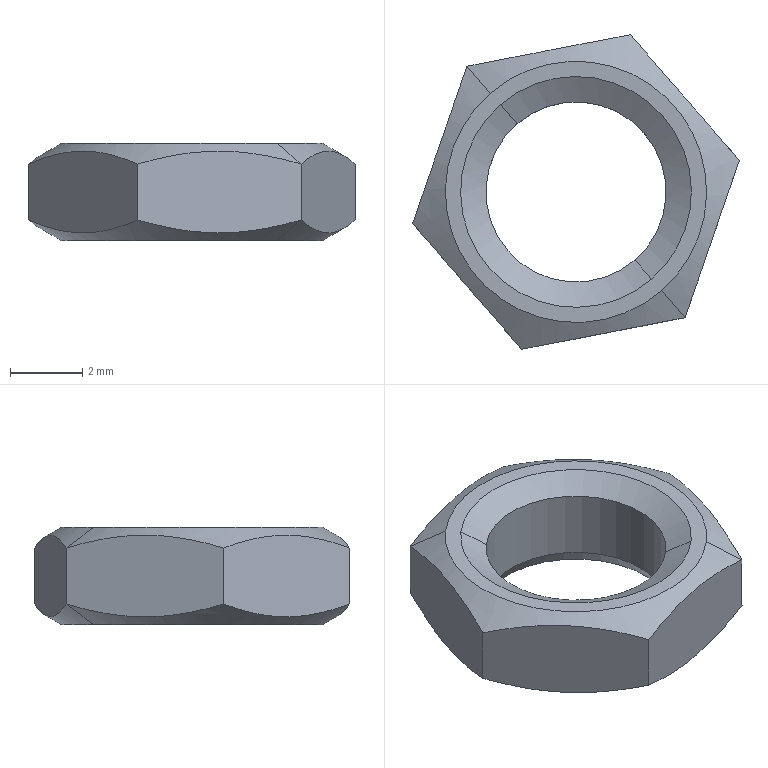Component | SolidWorks | HexThinNutGBT6172.1-M5-1 | 1 solid | 18 faces | box 9.07 x 8.73 x 2.7 mm | volume 88 mm3 | cone 8 | plane 8 | cylinder 2 | commonest cylinder face diameters 5 x2 | material Purchased Part
STEP:
#1=CARTESIAN_POINT('',(-3.125,-0.3253,-0.9055));
#2=VERTEX_POINT('',#1);
#3=CARTESIAN_POINT('',(-2.938,-0.5409,-0.9055));
#4=VERTEX_POINT('',#3);
#5=CARTESIAN_POINT('',(-3.031,-0.4331,-0.9055));
#6=DIRECTION('',(0.,0.,-1.));
#7=DIRECTION('',(0.6555,-0.7552,0.));
#8=AXIS2_PLACEMENT_3D('',#5,#6,#7);
#9=CIRCLE('',#8,0.1427);
#10=EDGE_CURVE('',#2,#4,#9,.T.);
#11=ORIENTED_EDGE('',*,*,#10,.F.);
#12=CARTESIAN_POINT('',(-3.151,-0.2957,-0.8829));
#13=VERTEX_POINT('',#12);
#14=CARTESIAN_POINT('',(-3.151,-0.2956,-0.8828));
#15=DIRECTION('',(-0.5676,0.654,0.5));
#16=VECTOR('',#15,39.37);
#17=LINE('',#14,#16);
#18=EDGE_CURVE('',#2,#13,#17,.T.);
#19=ORIENTED_EDGE('',*,*,#18,.T.);
#20=CARTESIAN_POINT('',(-2.972,-0.2612,-0.8829));
#21=VERTEX_POINT('',#20);
#22=CARTESIAN_POINT('',(-3.151,-0.2957,-0.8829));
#23=CARTESIAN_POINT('',(-3.122,-0.2901,-0.8915));
#24=CARTESIAN_POINT('',(-3.092,-0.2844,-0.897));
#25=CARTESIAN_POINT('',(-3.046,-0.2756,-0.897));
#26=CARTESIAN_POINT('',(-3.031,-0.2726,-0.8957));
#27=CARTESIAN_POINT('',(-3.001,-0.2669,-0.8908));
#28=CARTESIAN_POINT('',(-2.987,-0.264,-0.8872));
#29=CARTESIAN_POINT('',(-2.972,-0.2612,-0.8829));
#30=B_SPLINE_CURVE_WITH_KNOTS('',3,(#22,#23,#24,#25,#26,#27,#28,#29),.UNSPECIFIED.,.F.,.F.,(4,2,2,4),(0.,0.002332,0.003499,0.004665),.UNSPECIFIED.);
#31=EDGE_CURVE('',#13,#21,#30,.T.);
#32=ORIENTED_EDGE('',*,*,#31,.T.);
#33=CARTESIAN_POINT('',(-2.853,-0.3985,-0.8829));
#34=VERTEX_POINT('',#33);
#35=CARTESIAN_POINT('',(-2.972,-0.2612,-0.8829));
#36=CARTESIAN_POINT('',(-2.953,-0.2836,-0.8915));
#37=CARTESIAN_POINT('',(-2.933,-0.3064,-0.897));
#38=CARTESIAN_POINT('',(-2.903,-0.3414,-0.897));
#39=CARTESIAN_POINT('',(-2.892,-0.3531,-0.8957));
#40=CARTESIAN_POINT('',(-2.873,-0.376,-0.8908));
#41=CARTESIAN_POINT('',(-2.863,-0.3873,-0.8872));
#42=CARTESIAN_POINT('',(-2.853,-0.3985,-0.8829));
#43=B_SPLINE_CURVE_WITH_KNOTS('',3,(#35,#36,#37,#38,#39,#40,#41,#42),.UNSPECIFIED.,.F.,.F.,(4,2,2,4),(0.,0.002332,0.003499,0.004665),.UNSPECIFIED.);
#44=EDGE_CURVE('',#21,#34,#43,.T.);
#45=ORIENTED_EDGE('',*,*,#44,.T.);
#46=CARTESIAN_POINT('',(-2.912,-0.5704,-0.8829));
#47=VERTEX_POINT('',#46);
#48=CARTESIAN_POINT('',(-2.853,-0.3985,-0.8829));
#49=CARTESIAN_POINT('',(-2.863,-0.4266,-0.8915));
#50=CARTESIAN_POINT('',(-2.872,-0.4551,-0.897));
#51=CARTESIAN_POINT('',(-2.888,-0.4989,-0.897));
#52=CARTESIAN_POINT('',(-2.893,-0.5135,-0.8957));
#53=CARTESIAN_POINT('',(-2.903,-0.5422,-0.8908));
#54=CARTESIAN_POINT('',(-2.907,-0.5564,-0.8872));
#55=CARTESIAN_POINT('',(-2.912,-0.5704,-0.8829));
#56=B_SPLINE_CURVE_WITH_KNOTS('',3,(#48,#49,#50,#51,#52,#53,#54,#55),.UNSPECIFIED.,.F.,.F.,(4,2,2,4),(0.,0.002332,0.003499,0.004665),.UNSPECIFIED.);
#57=EDGE_CURVE('',#34,#47,#56,.T.);
#58=ORIENTED_EDGE('',*,*,#57,.T.);
#59=CARTESIAN_POINT('',(-2.912,-0.5706,-0.8828));
#60=DIRECTION('',(0.5676,-0.654,0.5));
#61=VECTOR('',#60,39.37);
#62=LINE('',#59,#61);
#63=EDGE_CURVE('',#4,#47,#62,.T.);
#64=ORIENTED_EDGE('',*,*,#63,.F.);
#65=EDGE_LOOP('',(#11,#19,#32,#45,#58,#64));
#66=FACE_OUTER_BOUND('',#65,.T.);
#67=CARTESIAN_POINT('',(-3.031,-0.4331,-0.8828));
#68=DIRECTION('',(0.,0.,1.));
#69=DIRECTION('',(0.6555,-0.7552,0.));
#70=AXIS2_PLACEMENT_3D('',#67,#68,#69);
#71=CONICAL_SURFACE('',#70,0.1821,1.047);
#72=ADVANCED_FACE('',(#66),#71,.T.);
#73=CARTESIAN_POINT('',(-2.967,-0.5074,-0.8903));
#74=VERTEX_POINT('',#73);
#75=CARTESIAN_POINT('',(-3.096,-0.3587,-0.8903));
#76=VERTEX_POINT('',#75);
#77=CARTESIAN_POINT('',(-3.031,-0.4331,-0.8903));
#78=DIRECTION('',(0.,0.,-1.));
#79=DIRECTION('',(-0.6555,0.7552,0.));
#80=AXIS2_PLACEMENT_3D('',#77,#78,#79);
#81=CIRCLE('',#80,0.09843);
#82=EDGE_CURVE('',#74,#76,#81,.T.);
#83=ORIENTED_EDGE('',*,*,#82,.F.);
#84=CARTESIAN_POINT('',(-2.961,-0.514,-0.9055));
#85=VERTEX_POINT('',#84);
#86=CARTESIAN_POINT('',(-2.964,-0.5103,-0.897));
#87=DIRECTION('',(0.3277,-0.3776,-0.866));
#88=VECTOR('',#87,39.37);
#89=LINE('',#86,#88);
#90=EDGE_CURVE('',#74,#85,#89,.T.);
#91=ORIENTED_EDGE('',*,*,#90,.T.);
#92=CARTESIAN_POINT('',(-3.102,-0.3521,-0.9055));
#93=VERTEX_POINT('',#92);
#94=CARTESIAN_POINT('',(-3.031,-0.4331,-0.9055));
#95=DIRECTION('',(0.,0.,1.));
#96=DIRECTION('',(-0.6555,0.7552,0.));
#97=AXIS2_PLACEMENT_3D('',#94,#95,#96);
#98=CIRCLE('',#97,0.1072);
#99=EDGE_CURVE('',#93,#85,#98,.T.);
#100=ORIENTED_EDGE('',*,*,#99,.F.);
#101=CARTESIAN_POINT('',(-3.099,-0.3558,-0.897));
#102=DIRECTION('',(-0.3277,0.3776,-0.866));
#103=VECTOR('',#102,39.37);
#104=LINE('',#101,#103);
#105=EDGE_CURVE('',#76,#93,#104,.T.);
#106=ORIENTED_EDGE('',*,*,#105,.F.);
#107=EDGE_LOOP('',(#83,#91,#100,#106));
#108=FACE_OUTER_BOUND('',#107,.T.);
#109=CARTESIAN_POINT('',(-3.031,-0.4331,-0.897));
#110=DIRECTION('',(0.,0.,-1.));
#111=DIRECTION('',(-0.6555,0.7552,0.));
#112=AXIS2_PLACEMENT_3D('',#109,#110,#111);
#113=CONICAL_SURFACE('',#112,0.1023,0.5236);
#114=ADVANCED_FACE('',(#108),#113,.F.);
#115=ORIENTED_EDGE('',*,*,#82,.T.);
#116=CARTESIAN_POINT('',(-3.096,-0.3587,-0.8152));
#117=VERTEX_POINT('',#116);
#118=CARTESIAN_POINT('',(-3.096,-0.3587,-0.9055));
#119=DIRECTION('',(0.,0.,1.));
#120=VECTOR('',#119,39.37);
#121=LINE('',#118,#120);
#122=EDGE_CURVE('',#76,#117,#121,.T.);
#123=ORIENTED_EDGE('',*,*,#122,.T.);
#124=CARTESIAN_POINT('',(-2.967,-0.5074,-0.8152));
#125=VERTEX_POINT('',#124);
#126=CARTESIAN_POINT('',(-3.031,-0.4331,-0.8152));
#127=DIRECTION('',(0.,0.,-1.));
#128=DIRECTION('',(0.6555,-0.7552,0.));
#129=AXIS2_PLACEMENT_3D('',#126,#127,#128);
#130=CIRCLE('',#129,0.09843);
#131=EDGE_CURVE('',#125,#117,#130,.T.);
#132=ORIENTED_EDGE('',*,*,#131,.F.);
#133=CARTESIAN_POINT('',(-2.967,-0.5074,-0.9055));
#134=DIRECTION('',(0.,0.,1.));
#135=VECTOR('',#134,39.37);
#136=LINE('',#133,#135);
#137=EDGE_CURVE('',#74,#125,#136,.T.);
#138=ORIENTED_EDGE('',*,*,#137,.F.);
#139=EDGE_LOOP('',(#115,#123,#132,#138));
#140=FACE_OUTER_BOUND('',#139,.T.);
#141=CARTESIAN_POINT('',(-3.031,-0.4331,-0.9055));
#142=DIRECTION('',(0.,0.,1.));
#143=DIRECTION('',(0.6555,-0.7552,0.));
#144=AXIS2_PLACEMENT_3D('',#141,#142,#143);
#145=CYLINDRICAL_SURFACE('',#144,0.09843);
#146=ADVANCED_FACE('',(#140),#145,.F.);
#147=CARTESIAN_POINT('',(-3.125,-0.3253,-0.7992));
#148=VERTEX_POINT('',#147);
#149=CARTESIAN_POINT('',(-2.938,-0.5409,-0.7992));
#150=VERTEX_POINT('',#149);
#151=CARTESIAN_POINT('',(-3.031,-0.4331,-0.7992));
#152=DIRECTION('',(0.,0.,-1.));
#153=DIRECTION('',(-0.6555,0.7552,0.));
#154=AXIS2_PLACEMENT_3D('',#151,#152,#153);
#155=CIRCLE('',#154,0.1427);
#156=EDGE_CURVE('',#148,#150,#155,.T.);
#157=ORIENTED_EDGE('',*,*,#156,.T.);
#158=CARTESIAN_POINT('',(-2.912,-0.5704,-0.8218));
#159=VERTEX_POINT('',#158);
#160=CARTESIAN_POINT('',(-2.912,-0.5706,-0.8219));
#161=DIRECTION('',(0.5676,-0.654,-0.5));
#162=VECTOR('',#161,39.37);
#163=LINE('',#160,#162);
#164=EDGE_CURVE('',#150,#159,#163,.T.);
#165=ORIENTED_EDGE('',*,*,#164,.T.);
#166=CARTESIAN_POINT('',(-2.853,-0.3985,-0.8218));
#167=VERTEX_POINT('',#166);
#168=CARTESIAN_POINT('',(-2.853,-0.3985,-0.8218));
#169=CARTESIAN_POINT('',(-2.863,-0.4266,-0.8132));
#170=CARTESIAN_POINT('',(-2.872,-0.4551,-0.8078));
#171=CARTESIAN_POINT('',(-2.888,-0.4989,-0.8077));
#172=CARTESIAN_POINT('',(-2.893,-0.5135,-0.8091));
#173=CARTESIAN_POINT('',(-2.903,-0.5422,-0.814));
#174=CARTESIAN_POINT('',(-2.907,-0.5564,-0.8175));
#175=CARTESIAN_POINT('',(-2.912,-0.5704,-0.8218));
#176=B_SPLINE_CURVE_WITH_KNOTS('',3,(#168,#169,#170,#171,#172,#173,#174,#175),.UNSPECIFIED.,.F.,.F.,(4,2,2,4),(0.,0.002332,0.003499,0.004665),.UNSPECIFIED.);
#177=EDGE_CURVE('',#167,#159,#176,.T.);
#178=ORIENTED_EDGE('',*,*,#177,.F.);
#179=CARTESIAN_POINT('',(-2.972,-0.2612,-0.8218));
#180=VERTEX_POINT('',#179);
#181=CARTESIAN_POINT('',(-2.972,-0.2612,-0.8218));
#182=CARTESIAN_POINT('',(-2.953,-0.2836,-0.8132));
#183=CARTESIAN_POINT('',(-2.933,-0.3064,-0.8078));
#184=CARTESIAN_POINT('',(-2.903,-0.3414,-0.8077));
#185=CARTESIAN_POINT('',(-2.892,-0.3531,-0.8091));
#186=CARTESIAN_POINT('',(-2.873,-0.376,-0.814));
#187=CARTESIAN_POINT('',(-2.863,-0.3873,-0.8175));
#188=CARTESIAN_POINT('',(-2.853,-0.3985,-0.8218));
#189=B_SPLINE_CURVE_WITH_KNOTS('',3,(#181,#182,#183,#184,#185,#186,#187,#188),.UNSPECIFIED.,.F.,.F.,(4,2,2,4),(0.,0.002332,0.003499,0.004665),.UNSPECIFIED.);
#190=EDGE_CURVE('',#180,#167,#189,.T.);
#191=ORIENTED_EDGE('',*,*,#190,.F.);
#192=CARTESIAN_POINT('',(-3.151,-0.2957,-0.8218));
#193=VERTEX_POINT('',#192);
#194=CARTESIAN_POINT('',(-3.151,-0.2957,-0.8218));
#195=CARTESIAN_POINT('',(-3.122,-0.2901,-0.8132));
#196=CARTESIAN_POINT('',(-3.092,-0.2844,-0.8078));
#197=CARTESIAN_POINT('',(-3.046,-0.2756,-0.8077));
#198=CARTESIAN_POINT('',(-3.031,-0.2726,-0.8091));
#199=CARTESIAN_POINT('',(-3.001,-0.2669,-0.814));
#200=CARTESIAN_POINT('',(-2.987,-0.264,-0.8175));
#201=CARTESIAN_POINT('',(-2.972,-0.2612,-0.8218));
#202=B_SPLINE_CURVE_WITH_KNOTS('',3,(#194,#195,#196,#197,#198,#199,#200,#201),.UNSPECIFIED.,.F.,.F.,(4,2,2,4),(0.,0.002332,0.003499,0.004665),.UNSPECIFIED.);
#203=EDGE_CURVE('',#193,#180,#202,.T.);
#204=ORIENTED_EDGE('',*,*,#203,.F.);
#205=CARTESIAN_POINT('',(-3.151,-0.2956,-0.8219));
#206=DIRECTION('',(-0.5676,0.654,-0.5));
#207=VECTOR('',#206,39.37);
#208=LINE('',#205,#207);
#209=EDGE_CURVE('',#148,#193,#208,.T.);
#210=ORIENTED_EDGE('',*,*,#209,.F.);
#211=EDGE_LOOP('',(#157,#165,#178,#191,#204,#210));
#212=FACE_OUTER_BOUND('',#211,.T.);
#213=CARTESIAN_POINT('',(-3.031,-0.4331,-0.8219));
#214=DIRECTION('',(0.,0.,-1.));
#215=DIRECTION('',(-0.6555,0.7552,0.));
#216=AXIS2_PLACEMENT_3D('',#213,#214,#215);
#217=CONICAL_SURFACE('',#216,0.1821,1.047);
#218=ADVANCED_FACE('',(#212),#217,.T.);
#219=ORIENTED_EDGE('',*,*,#131,.T.);
#220=CARTESIAN_POINT('',(-3.114,-0.3378,-0.7992));
#221=VERTEX_POINT('',#220);
#222=CARTESIAN_POINT('',(-3.097,-0.3571,-0.814));
#223=DIRECTION('',(-0.5676,0.654,0.5));
#224=VECTOR('',#223,39.37);
#225=LINE('',#222,#224);
#226=EDGE_CURVE('',#117,#221,#225,.T.);
#227=ORIENTED_EDGE('',*,*,#226,.T.);
#228=CARTESIAN_POINT('',(-2.949,-0.5283,-0.7992));
#229=VERTEX_POINT('',#228);
#230=CARTESIAN_POINT('',(-3.031,-0.4331,-0.7992));
#231=DIRECTION('',(0.,0.,-1.));
#232=DIRECTION('',(-0.6555,0.7552,0.));
#233=AXIS2_PLACEMENT_3D('',#230,#231,#232);
#234=CIRCLE('',#233,0.1261);
#235=EDGE_CURVE('',#229,#221,#234,.T.);
#236=ORIENTED_EDGE('',*,*,#235,.F.);
#237=CARTESIAN_POINT('',(-2.966,-0.509,-0.814));
#238=DIRECTION('',(0.5676,-0.654,0.5));
#239=VECTOR('',#238,39.37);
#240=LINE('',#237,#239);
#241=EDGE_CURVE('',#125,#229,#240,.T.);
#242=ORIENTED_EDGE('',*,*,#241,.F.);
#243=EDGE_LOOP('',(#219,#227,#236,#242));
#244=FACE_OUTER_BOUND('',#243,.T.);
#245=CARTESIAN_POINT('',(-3.031,-0.4331,-0.814));
#246=DIRECTION('',(0.,0.,1.));
#247=DIRECTION('',(0.6555,-0.7552,0.));
#248=AXIS2_PLACEMENT_3D('',#245,#246,#247);
#249=CONICAL_SURFACE('',#248,0.1005,1.047);
#250=ADVANCED_FACE('',(#244),#249,.F.);
#251=CARTESIAN_POINT('',(-3.031,-0.4331,-0.9055));
#252=DIRECTION('',(0.,0.,-1.));
#253=DIRECTION('',(0.6555,-0.7552,0.));
#254=AXIS2_PLACEMENT_3D('',#251,#252,#253);
#255=CIRCLE('',#254,0.1427);
#256=EDGE_CURVE('',#4,#2,#255,.T.);
#257=ORIENTED_EDGE('',*,*,#256,.T.);
#258=ORIENTED_EDGE('',*,*,#10,.T.);
#259=EDGE_LOOP('',(#257,#258));
#260=FACE_OUTER_BOUND('',#259,.T.);
#261=ORIENTED_EDGE('',*,*,#99,.T.);
#262=CARTESIAN_POINT('',(-3.031,-0.4331,-0.9055));
#263=DIRECTION('',(0.,0.,1.));
#264=DIRECTION('',(-0.6555,0.7552,0.));
#265=AXIS2_PLACEMENT_3D('',#262,#263,#264);
#266=CIRCLE('',#265,0.1072);
#267=EDGE_CURVE('',#85,#93,#266,.T.);
#268=ORIENTED_EDGE('',*,*,#267,.T.);
#269=EDGE_LOOP('',(#261,#268));
#270=FACE_BOUND('',#269,.T.);
#271=CARTESIAN_POINT('',(-3.21,-0.4676,-0.9055));
#272=DIRECTION('',(0.,0.,-1.));
#273=DIRECTION('',(-0.6555,0.7552,0.));
#274=AXIS2_PLACEMENT_3D('',#271,#272,#273);
#275=PLANE('',#274);
#276=ADVANCED_FACE('',(#260,#270),#275,.T.);
#277=ORIENTED_EDGE('',*,*,#18,.F.);
#278=ORIENTED_EDGE('',*,*,#256,.F.);
#279=ORIENTED_EDGE('',*,*,#63,.T.);
#280=CARTESIAN_POINT('',(-3.091,-0.605,-0.8829));
#281=VERTEX_POINT('',#280);
#282=CARTESIAN_POINT('',(-2.912,-0.5704,-0.8829));
#283=CARTESIAN_POINT('',(-2.941,-0.576,-0.8915));
#284=CARTESIAN_POINT('',(-2.971,-0.5818,-0.897));
#285=CARTESIAN_POINT('',(-3.017,-0.5906,-0.897));
#286=CARTESIAN_POINT('',(-3.032,-0.5935,-0.8957));
#287=CARTESIAN_POINT('',(-3.062,-0.5993,-0.8908));
#288=CARTESIAN_POINT('',(-3.076,-0.6021,-0.8872));
#289=CARTESIAN_POINT('',(-3.091,-0.605,-0.8829));
#290=B_SPLINE_CURVE_WITH_KNOTS('',3,(#282,#283,#284,#285,#286,#287,#288,#289),.UNSPECIFIED.,.F.,.F.,(4,2,2,4),(0.,0.002332,0.003499,0.004665),.UNSPECIFIED.);
#291=EDGE_CURVE('',#47,#281,#290,.T.);
#292=ORIENTED_EDGE('',*,*,#291,.T.);
#293=CARTESIAN_POINT('',(-3.21,-0.4676,-0.8829));
#294=VERTEX_POINT('',#293);
#295=CARTESIAN_POINT('',(-3.091,-0.605,-0.8829));
#296=CARTESIAN_POINT('',(-3.11,-0.5825,-0.8915));
#297=CARTESIAN_POINT('',(-3.13,-0.5598,-0.897));
#298=CARTESIAN_POINT('',(-3.16,-0.5247,-0.897));
#299=CARTESIAN_POINT('',(-3.171,-0.5131,-0.8957));
#300=CARTESIAN_POINT('',(-3.19,-0.4902,-0.8908));
#301=CARTESIAN_POINT('',(-3.2,-0.4789,-0.8872));
#302=CARTESIAN_POINT('',(-3.21,-0.4676,-0.8829));
#303=B_SPLINE_CURVE_WITH_KNOTS('',3,(#295,#296,#297,#298,#299,#300,#301,#302),.UNSPECIFIED.,.F.,.F.,(4,2,2,4),(0.,0.002332,0.003499,0.004665),.UNSPECIFIED.);
#304=EDGE_CURVE('',#281,#294,#303,.T.);
#305=ORIENTED_EDGE('',*,*,#304,.T.);
#306=CARTESIAN_POINT('',(-3.21,-0.4676,-0.8829));
#307=CARTESIAN_POINT('',(-3.2,-0.4396,-0.8915));
#308=CARTESIAN_POINT('',(-3.191,-0.4111,-0.897));
#309=CARTESIAN_POINT('',(-3.175,-0.3672,-0.897));
#310=CARTESIAN_POINT('',(-3.17,-0.3526,-0.8957));
#311=CARTESIAN_POINT('',(-3.16,-0.324,-0.8908));
#312=CARTESIAN_POINT('',(-3.156,-0.3098,-0.8872));
#313=CARTESIAN_POINT('',(-3.151,-0.2957,-0.8829));
#314=B_SPLINE_CURVE_WITH_KNOTS('',3,(#306,#307,#308,#309,#310,#311,#312,#313),.UNSPECIFIED.,.F.,.F.,(4,2,2,4),(0.,0.002332,0.003499,0.004665),.UNSPECIFIED.);
#315=EDGE_CURVE('',#294,#13,#314,.T.);
#316=ORIENTED_EDGE('',*,*,#315,.T.);
#317=EDGE_LOOP('',(#277,#278,#279,#292,#305,#316));
#318=FACE_OUTER_BOUND('',#317,.T.);
#319=CARTESIAN_POINT('',(-3.031,-0.4331,-0.8828));
#320=DIRECTION('',(0.,0.,1.));
#321=DIRECTION('',(0.6555,-0.7552,0.));
#322=AXIS2_PLACEMENT_3D('',#319,#320,#321);
#323=CONICAL_SURFACE('',#322,0.1821,1.047);
#324=ADVANCED_FACE('',(#318),#323,.T.);
#325=ORIENTED_EDGE('',*,*,#90,.F.);
#326=CARTESIAN_POINT('',(-3.031,-0.4331,-0.8903));
#327=DIRECTION('',(0.,0.,-1.));
#328=DIRECTION('',(-0.6555,0.7552,0.));
#329=AXIS2_PLACEMENT_3D('',#326,#327,#328);
#330=CIRCLE('',#329,0.09843);
#331=EDGE_CURVE('',#76,#74,#330,.T.);
#332=ORIENTED_EDGE('',*,*,#331,.F.);
#333=ORIENTED_EDGE('',*,*,#105,.T.);
#334=ORIENTED_EDGE('',*,*,#267,.F.);
#335=EDGE_LOOP('',(#325,#332,#333,#334));
#336=FACE_OUTER_BOUND('',#335,.T.);
#337=CARTESIAN_POINT('',(-3.031,-0.4331,-0.897));
#338=DIRECTION('',(0.,0.,-1.));
#339=DIRECTION('',(-0.6555,0.7552,0.));
#340=AXIS2_PLACEMENT_3D('',#337,#338,#339);
#341=CONICAL_SURFACE('',#340,0.1023,0.5236);
#342=ADVANCED_FACE('',(#336),#341,.F.);
#343=ORIENTED_EDGE('',*,*,#57,.F.);
#344=CARTESIAN_POINT('',(-2.853,-0.3985,-0.9055));
#345=DIRECTION('',(0.,0.,1.));
#346=VECTOR('',#345,39.37);
#347=LINE('',#344,#346);
#348=EDGE_CURVE('',#34,#167,#347,.T.);
#349=ORIENTED_EDGE('',*,*,#348,.T.);
#350=ORIENTED_EDGE('',*,*,#177,.T.);
#351=CARTESIAN_POINT('',(-2.912,-0.5704,-0.9055));
#352=DIRECTION('',(0.,0.,-1.));
#353=VECTOR('',#352,39.37);
#354=LINE('',#351,#353);
#355=EDGE_CURVE('',#159,#47,#354,.T.);
#356=ORIENTED_EDGE('',*,*,#355,.T.);
#357=EDGE_LOOP('',(#343,#349,#350,#356));
#358=FACE_OUTER_BOUND('',#357,.T.);
#359=CARTESIAN_POINT('',(-2.912,-0.5704,-0.9055));
#360=DIRECTION('',(0.9453,-0.3263,0.));
#361=DIRECTION('',(0.3263,0.9453,0.));
#362=AXIS2_PLACEMENT_3D('',#359,#360,#361);
#363=PLANE('',#362);
#364=ADVANCED_FACE('',(#358),#363,.T.);
#365=ORIENTED_EDGE('',*,*,#44,.F.);
#366=CARTESIAN_POINT('',(-2.972,-0.2612,-0.9055));
#367=DIRECTION('',(0.,0.,1.));
#368=VECTOR('',#367,39.37);
#369=LINE('',#366,#368);
#370=EDGE_CURVE('',#21,#180,#369,.T.);
#371=ORIENTED_EDGE('',*,*,#370,.T.);
#372=ORIENTED_EDGE('',*,*,#190,.T.);
#373=ORIENTED_EDGE('',*,*,#348,.F.);
#374=EDGE_LOOP('',(#365,#371,#372,#373));
#375=FACE_OUTER_BOUND('',#374,.T.);
#376=CARTESIAN_POINT('',(-2.853,-0.3985,-0.9055));
#377=DIRECTION('',(0.7552,0.6555,0.));
#378=DIRECTION('',(0.,0.,1.));
#379=AXIS2_PLACEMENT_3D('',#376,#377,#378);
#380=PLANE('',#379);
#381=ADVANCED_FACE('',(#375),#380,.T.);
#382=ORIENTED_EDGE('',*,*,#31,.F.);
#383=CARTESIAN_POINT('',(-3.151,-0.2957,-0.9055));
#384=DIRECTION('',(0.,0.,1.));
#385=VECTOR('',#384,39.37);
#386=LINE('',#383,#385);
#387=EDGE_CURVE('',#13,#193,#386,.T.);
#388=ORIENTED_EDGE('',*,*,#387,.T.);
#389=ORIENTED_EDGE('',*,*,#203,.T.);
#390=ORIENTED_EDGE('',*,*,#370,.F.);
#391=EDGE_LOOP('',(#382,#388,#389,#390));
#392=FACE_OUTER_BOUND('',#391,.T.);
#393=CARTESIAN_POINT('',(-2.972,-0.2612,-0.9055));
#394=DIRECTION('',(-0.19,0.9818,0.));
#395=DIRECTION('',(-0.9818,-0.19,0.));
#396=AXIS2_PLACEMENT_3D('',#393,#394,#395);
#397=PLANE('',#396);
#398=ADVANCED_FACE('',(#392),#397,.T.);
#399=ORIENTED_EDGE('',*,*,#315,.F.);
#400=CARTESIAN_POINT('',(-3.21,-0.4676,-0.8218));
#401=VERTEX_POINT('',#400);
#402=CARTESIAN_POINT('',(-3.21,-0.4676,-0.9055));
#403=DIRECTION('',(0.,0.,1.));
#404=VECTOR('',#403,39.37);
#405=LINE('',#402,#404);
#406=EDGE_CURVE('',#294,#401,#405,.T.);
#407=ORIENTED_EDGE('',*,*,#406,.T.);
#408=CARTESIAN_POINT('',(-3.21,-0.4676,-0.8218));
#409=CARTESIAN_POINT('',(-3.2,-0.4396,-0.8132));
#410=CARTESIAN_POINT('',(-3.191,-0.4111,-0.8078));
#411=CARTESIAN_POINT('',(-3.175,-0.3672,-0.8077));
#412=CARTESIAN_POINT('',(-3.17,-0.3526,-0.8091));
#413=CARTESIAN_POINT('',(-3.16,-0.324,-0.814));
#414=CARTESIAN_POINT('',(-3.156,-0.3098,-0.8175));
#415=CARTESIAN_POINT('',(-3.151,-0.2957,-0.8218));
#416=B_SPLINE_CURVE_WITH_KNOTS('',3,(#408,#409,#410,#411,#412,#413,#414,#415),.UNSPECIFIED.,.F.,.F.,(4,2,2,4),(0.,0.002332,0.003499,0.004665),.UNSPECIFIED.);
#417=EDGE_CURVE('',#401,#193,#416,.T.);
#418=ORIENTED_EDGE('',*,*,#417,.T.);
#419=ORIENTED_EDGE('',*,*,#387,.F.);
#420=EDGE_LOOP('',(#399,#407,#418,#419));
#421=FACE_OUTER_BOUND('',#420,.T.);
#422=CARTESIAN_POINT('',(-3.151,-0.2957,-0.9055));
#423=DIRECTION('',(-0.9453,0.3263,0.));
#424=DIRECTION('',(-0.3263,-0.9453,0.));
#425=AXIS2_PLACEMENT_3D('',#422,#423,#424);
#426=PLANE('',#425);
#427=ADVANCED_FACE('',(#421),#426,.T.);
#428=ORIENTED_EDGE('',*,*,#304,.F.);
#429=CARTESIAN_POINT('',(-3.091,-0.605,-0.8218));
#430=VERTEX_POINT('',#429);
#431=CARTESIAN_POINT('',(-3.091,-0.605,-0.9055));
#432=DIRECTION('',(0.,0.,1.));
#433=VECTOR('',#432,39.37);
#434=LINE('',#431,#433);
#435=EDGE_CURVE('',#281,#430,#434,.T.);
#436=ORIENTED_EDGE('',*,*,#435,.T.);
#437=CARTESIAN_POINT('',(-3.091,-0.605,-0.8218));
#438=CARTESIAN_POINT('',(-3.11,-0.5825,-0.8132));
#439=CARTESIAN_POINT('',(-3.13,-0.5598,-0.8078));
#440=CARTESIAN_POINT('',(-3.16,-0.5247,-0.8077));
#441=CARTESIAN_POINT('',(-3.171,-0.5131,-0.8091));
#442=CARTESIAN_POINT('',(-3.19,-0.4902,-0.814));
#443=CARTESIAN_POINT('',(-3.2,-0.4789,-0.8175));
#444=CARTESIAN_POINT('',(-3.21,-0.4676,-0.8218));
#445=B_SPLINE_CURVE_WITH_KNOTS('',3,(#437,#438,#439,#440,#441,#442,#443,#444),.UNSPECIFIED.,.F.,.F.,(4,2,2,4),(0.,0.002332,0.003499,0.004665),.UNSPECIFIED.);
#446=EDGE_CURVE('',#430,#401,#445,.T.);
#447=ORIENTED_EDGE('',*,*,#446,.T.);
#448=ORIENTED_EDGE('',*,*,#406,.F.);
#449=EDGE_LOOP('',(#428,#436,#447,#448));
#450=FACE_OUTER_BOUND('',#449,.T.);
#451=CARTESIAN_POINT('',(-3.21,-0.4676,-0.9055));
#452=DIRECTION('',(-0.7552,-0.6555,0.));
#453=DIRECTION('',(0.6555,-0.7552,0.));
#454=AXIS2_PLACEMENT_3D('',#451,#452,#453);
#455=PLANE('',#454);
#456=ADVANCED_FACE('',(#450),#455,.T.);
#457=ORIENTED_EDGE('',*,*,#291,.F.);
#458=ORIENTED_EDGE('',*,*,#355,.F.);
#459=CARTESIAN_POINT('',(-2.912,-0.5704,-0.8218));
#460=CARTESIAN_POINT('',(-2.941,-0.576,-0.8132));
#461=CARTESIAN_POINT('',(-2.971,-0.5818,-0.8078));
#462=CARTESIAN_POINT('',(-3.017,-0.5906,-0.8077));
#463=CARTESIAN_POINT('',(-3.032,-0.5935,-0.8091));
#464=CARTESIAN_POINT('',(-3.062,-0.5993,-0.814));
#465=CARTESIAN_POINT('',(-3.076,-0.6021,-0.8175));
#466=CARTESIAN_POINT('',(-3.091,-0.605,-0.8218));
#467=B_SPLINE_CURVE_WITH_KNOTS('',3,(#459,#460,#461,#462,#463,#464,#465,#466),.UNSPECIFIED.,.F.,.F.,(4,2,2,4),(0.,0.002332,0.003499,0.004665),.UNSPECIFIED.);
#468=EDGE_CURVE('',#159,#430,#467,.T.);
#469=ORIENTED_EDGE('',*,*,#468,.T.);
#470=ORIENTED_EDGE('',*,*,#435,.F.);
#471=EDGE_LOOP('',(#457,#458,#469,#470));
#472=FACE_OUTER_BOUND('',#471,.T.);
#473=CARTESIAN_POINT('',(-3.091,-0.605,-0.9055));
#474=DIRECTION('',(0.19,-0.9818,0.));
#475=DIRECTION('',(0.9818,0.19,0.));
#476=AXIS2_PLACEMENT_3D('',#473,#474,#475);
#477=PLANE('',#476);
#478=ADVANCED_FACE('',(#472),#477,.T.);
#479=ORIENTED_EDGE('',*,*,#122,.F.);
#480=ORIENTED_EDGE('',*,*,#331,.T.);
#481=ORIENTED_EDGE('',*,*,#137,.T.);
#482=CARTESIAN_POINT('',(-3.031,-0.4331,-0.8152));
#483=DIRECTION('',(0.,0.,-1.));
#484=DIRECTION('',(0.6555,-0.7552,0.));
#485=AXIS2_PLACEMENT_3D('',#482,#483,#484);
#486=CIRCLE('',#485,0.09843);
#487=EDGE_CURVE('',#117,#125,#486,.T.);
#488=ORIENTED_EDGE('',*,*,#487,.F.);
#489=EDGE_LOOP('',(#479,#480,#481,#488));
#490=FACE_OUTER_BOUND('',#489,.T.);
#491=CARTESIAN_POINT('',(-3.031,-0.4331,-0.9055));
#492=DIRECTION('',(0.,0.,1.));
#493=DIRECTION('',(0.6555,-0.7552,0.));
#494=AXIS2_PLACEMENT_3D('',#491,#492,#493);
#495=CYLINDRICAL_SURFACE('',#494,0.09843);
#496=ADVANCED_FACE('',(#490),#495,.F.);
#497=ORIENTED_EDGE('',*,*,#164,.F.);
#498=CARTESIAN_POINT('',(-3.031,-0.4331,-0.7992));
#499=DIRECTION('',(0.,0.,-1.));
#500=DIRECTION('',(-0.6555,0.7552,0.));
#501=AXIS2_PLACEMENT_3D('',#498,#499,#500);
#502=CIRCLE('',#501,0.1427);
#503=EDGE_CURVE('',#150,#148,#502,.T.);
#504=ORIENTED_EDGE('',*,*,#503,.T.);
#505=ORIENTED_EDGE('',*,*,#209,.T.);
#506=ORIENTED_EDGE('',*,*,#417,.F.);
#507=ORIENTED_EDGE('',*,*,#446,.F.);
#508=ORIENTED_EDGE('',*,*,#468,.F.);
#509=EDGE_LOOP('',(#497,#504,#505,#506,#507,#508));
#510=FACE_OUTER_BOUND('',#509,.T.);
#511=CARTESIAN_POINT('',(-3.031,-0.4331,-0.8219));
#512=DIRECTION('',(0.,0.,-1.));
#513=DIRECTION('',(-0.6555,0.7552,0.));
#514=AXIS2_PLACEMENT_3D('',#511,#512,#513);
#515=CONICAL_SURFACE('',#514,0.1821,1.047);
#516=ADVANCED_FACE('',(#510),#515,.T.);
#517=ORIENTED_EDGE('',*,*,#226,.F.);
#518=ORIENTED_EDGE('',*,*,#487,.T.);
#519=ORIENTED_EDGE('',*,*,#241,.T.);
#520=CARTESIAN_POINT('',(-3.031,-0.4331,-0.7992));
#521=DIRECTION('',(0.,0.,-1.));
#522=DIRECTION('',(-0.6555,0.7552,0.));
#523=AXIS2_PLACEMENT_3D('',#520,#521,#522);
#524=CIRCLE('',#523,0.1261);
#525=EDGE_CURVE('',#221,#229,#524,.T.);
#526=ORIENTED_EDGE('',*,*,#525,.F.);
#527=EDGE_LOOP('',(#517,#518,#519,#526));
#528=FACE_OUTER_BOUND('',#527,.T.);
#529=CARTESIAN_POINT('',(-3.031,-0.4331,-0.814));
#530=DIRECTION('',(0.,0.,1.));
#531=DIRECTION('',(0.6555,-0.7552,0.));
#532=AXIS2_PLACEMENT_3D('',#529,#530,#531);
#533=CONICAL_SURFACE('',#532,0.1005,1.047);
#534=ADVANCED_FACE('',(#528),#533,.F.);
#535=ORIENTED_EDGE('',*,*,#156,.F.);
#536=ORIENTED_EDGE('',*,*,#503,.F.);
#537=EDGE_LOOP('',(#535,#536));
#538=FACE_OUTER_BOUND('',#537,.T.);
#539=ORIENTED_EDGE('',*,*,#235,.T.);
#540=ORIENTED_EDGE('',*,*,#525,.T.);
#541=EDGE_LOOP('',(#539,#540));
#542=FACE_BOUND('',#541,.T.);
#543=CARTESIAN_POINT('',(-3.21,-0.4676,-0.7992));
#544=DIRECTION('',(0.,0.,-1.));
#545=DIRECTION('',(-0.6555,0.7552,0.));
#546=AXIS2_PLACEMENT_3D('',#543,#544,#545);
#547=PLANE('',#546);
#548=ADVANCED_FACE('',(#538,#542),#547,.F.);
#549=CLOSED_SHELL('',(#72,#114,#146,#218,#250,#276,#324,#342,#364,#381,#398,#427,#456,#478,#496,#516,#534,#548));
#550=MANIFOLD_SOLID_BREP('',#549);
#551=CARTESIAN_POINT('',(0.,0.,0.));
#552=DIRECTION('',(0.,0.,1.));
#553=DIRECTION('',(1.,0.,0.));
#554=AXIS2_PLACEMENT_3D('',#551,#552,#553);
#555=(LENGTH_UNIT()NAMED_UNIT(*)SI_UNIT($,.METRE.));
#556=LENGTH_MEASURE_WITH_UNIT(LENGTH_MEASURE(0.0254),#555);
#557=DIMENSIONAL_EXPONENTS(1.,0.,0.,0.,0.,0.,0.);
#558=(CONVERSION_BASED_UNIT('',#556)LENGTH_UNIT()NAMED_UNIT(#557));
#559=UNCERTAINTY_MEASURE_WITH_UNIT(LENGTH_MEASURE(0.00001),#558,'','');
#560=(NAMED_UNIT(*)PLANE_ANGLE_UNIT()SI_UNIT($,.RADIAN.));
#561=(NAMED_UNIT(*)SI_UNIT($,.STERADIAN.)SOLID_ANGLE_UNIT());
#562=(GEOMETRIC_REPRESENTATION_CONTEXT(3)GLOBAL_UNCERTAINTY_ASSIGNED_CONTEXT((#559))GLOBAL_UNIT_ASSIGNED_CONTEXT((#558,#560,#561))REPRESENTATION_CONTEXT('',''));
#563=ADVANCED_BREP_SHAPE_REPRESENTATION('',(#550,#554),#562);
#564=COLOUR_RGB('',0.7922,0.8196,0.9333);
#565=FILL_AREA_STYLE_COLOUR('',#564);
#566=FILL_AREA_STYLE('',(#565));
#567=SURFACE_STYLE_FILL_AREA(#566);
#568=SURFACE_SIDE_STYLE('',(#567));
#569=SURFACE_STYLE_USAGE(.BOTH.,#568);
#570=PRESENTATION_STYLE_ASSIGNMENT((#569));
#571=STYLED_ITEM('',(#570),#550);
#572=PRESENTATION_LAYER_ASSIGNMENT('','',(#571));
#573=(LENGTH_UNIT()NAMED_UNIT(*)SI_UNIT($,.METRE.));
#574=LENGTH_MEASURE_WITH_UNIT(LENGTH_MEASURE(0.0254),#573);
#575=DIMENSIONAL_EXPONENTS(1.,0.,0.,0.,0.,0.,0.);
#576=(CONVERSION_BASED_UNIT('',#574)LENGTH_UNIT()NAMED_UNIT(#575));
#577=UNCERTAINTY_MEASURE_WITH_UNIT(LENGTH_MEASURE(0.00001),#576,'','');
#578=(NAMED_UNIT(*)PLANE_ANGLE_UNIT()SI_UNIT($,.RADIAN.));
#579=(NAMED_UNIT(*)SI_UNIT($,.STERADIAN.)SOLID_ANGLE_UNIT());
#580=(GEOMETRIC_REPRESENTATION_CONTEXT(3)GLOBAL_UNCERTAINTY_ASSIGNED_CONTEXT((#577))GLOBAL_UNIT_ASSIGNED_CONTEXT((#576,#578,#579))REPRESENTATION_CONTEXT('',''));
#581=MECHANICAL_DESIGN_GEOMETRIC_PRESENTATION_REPRESENTATION('',(#571),#580);